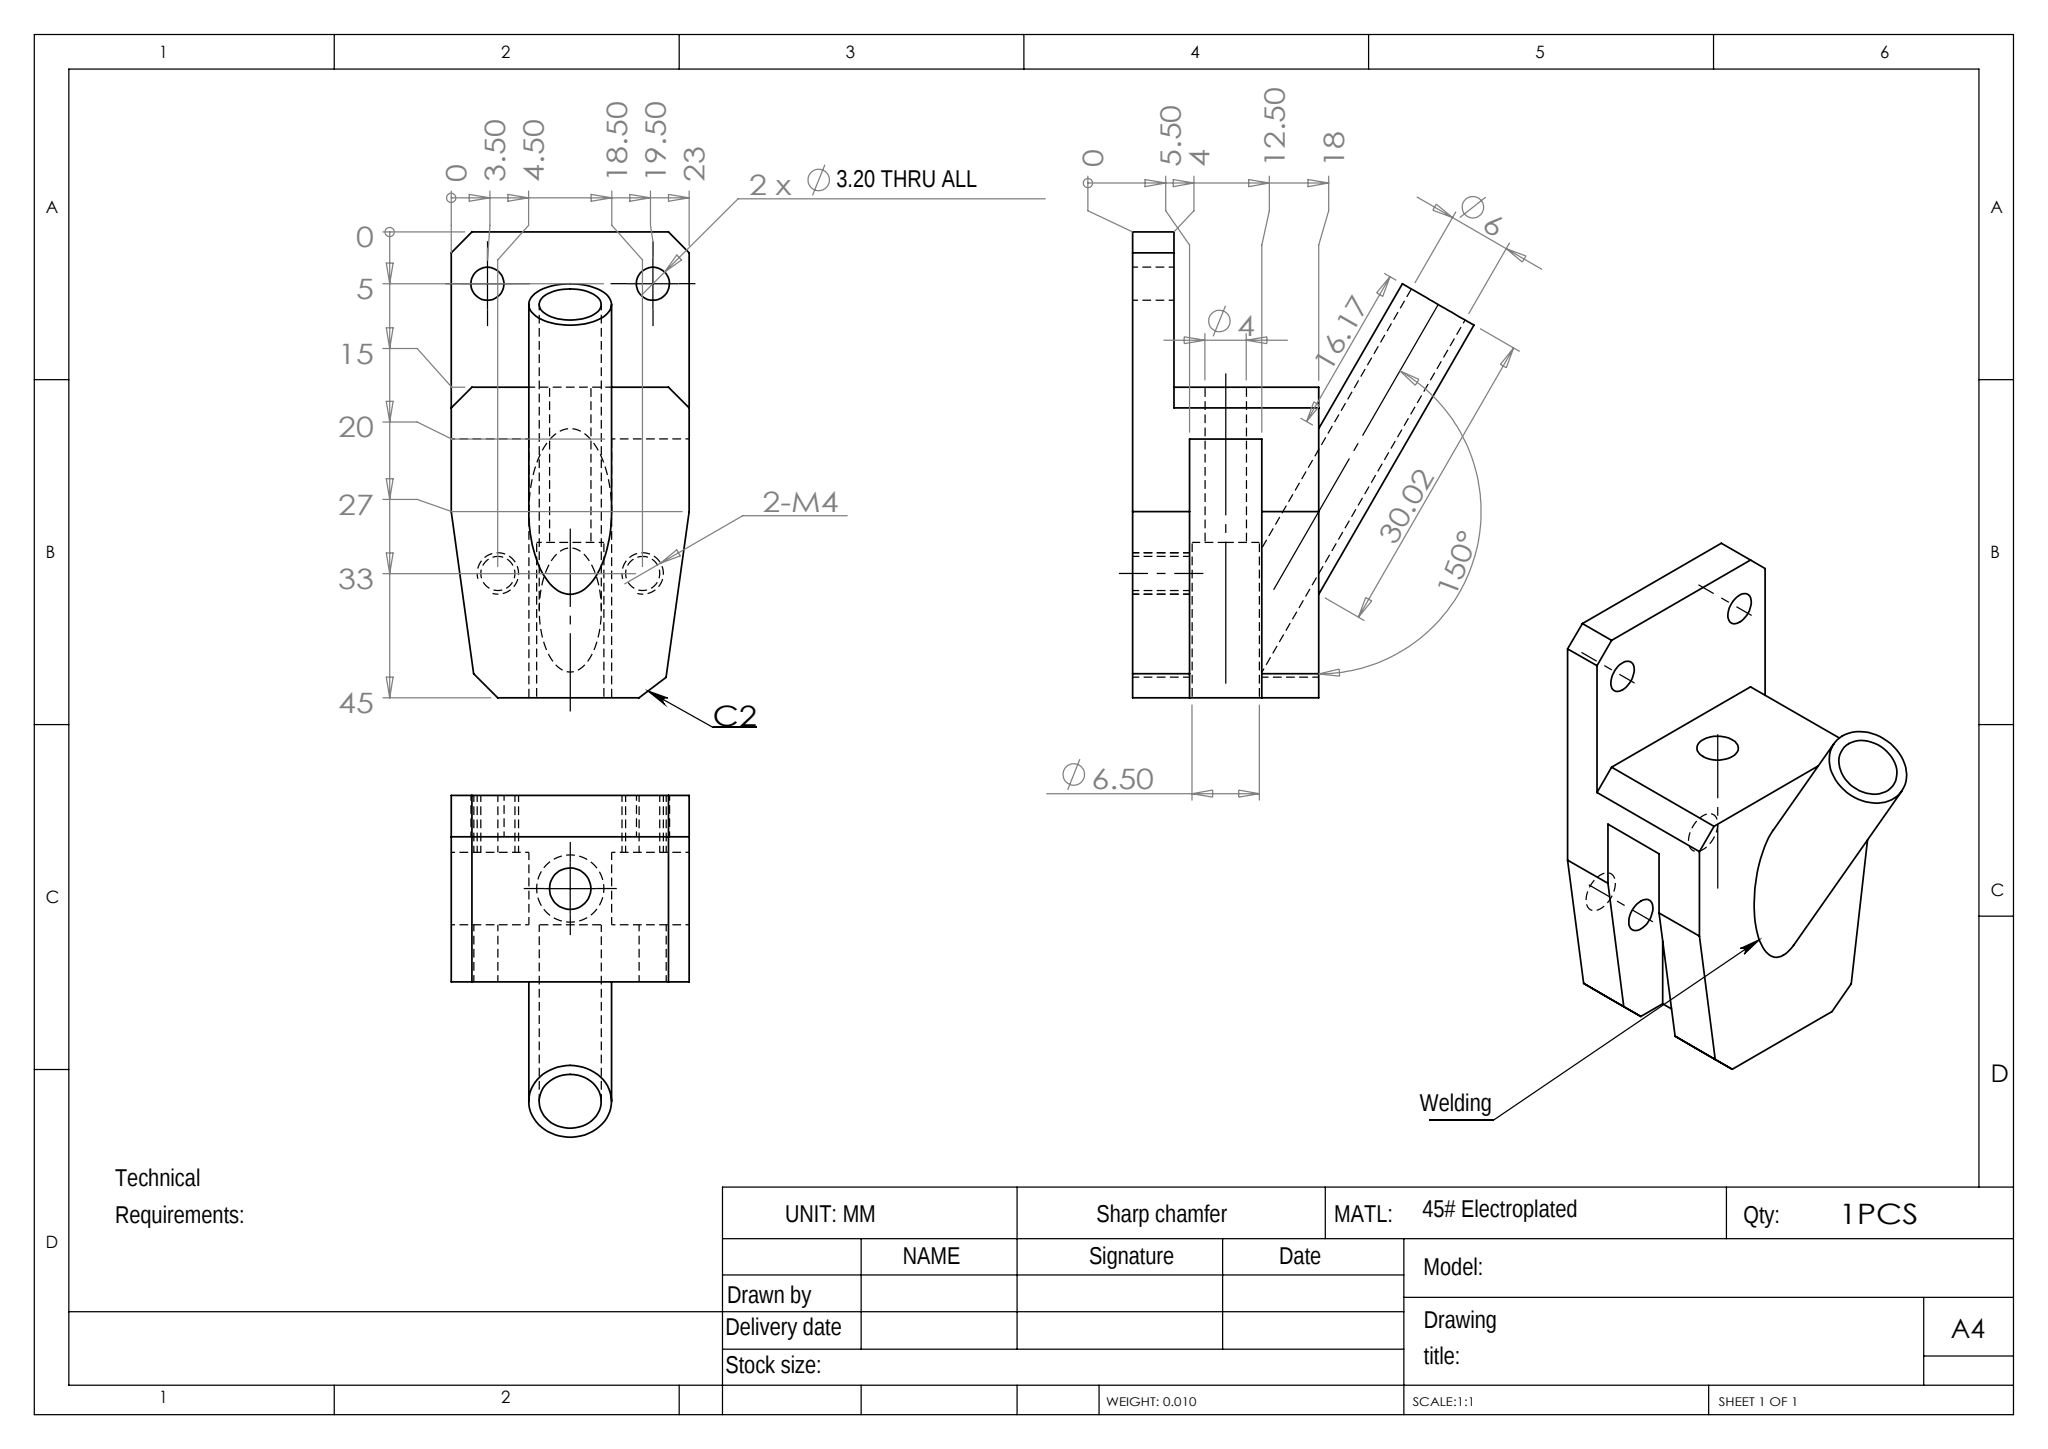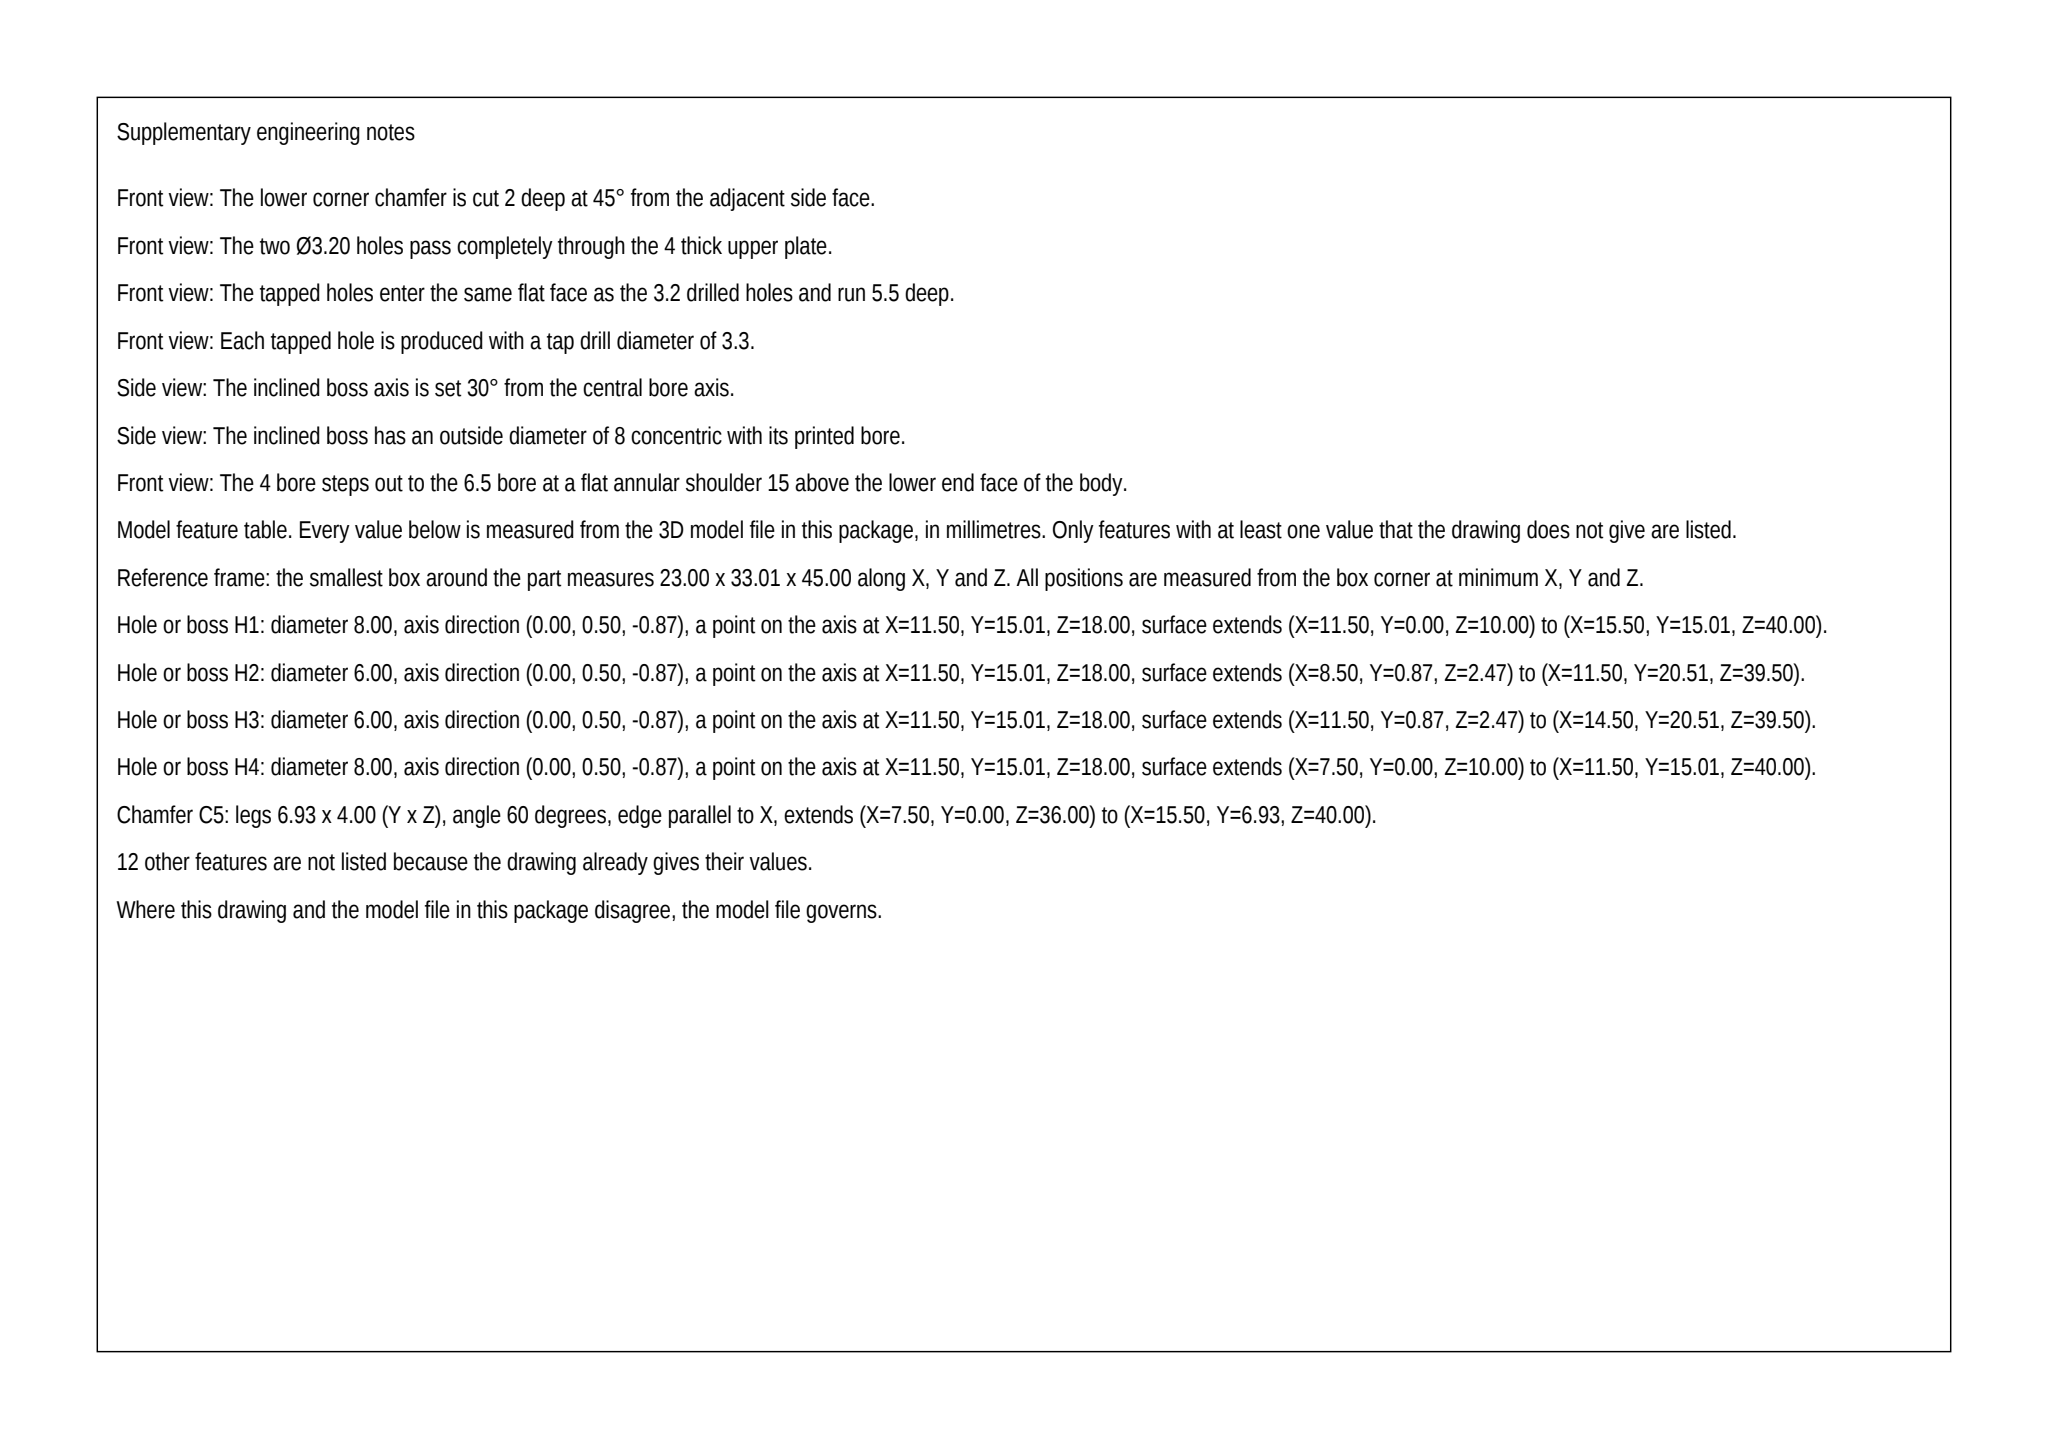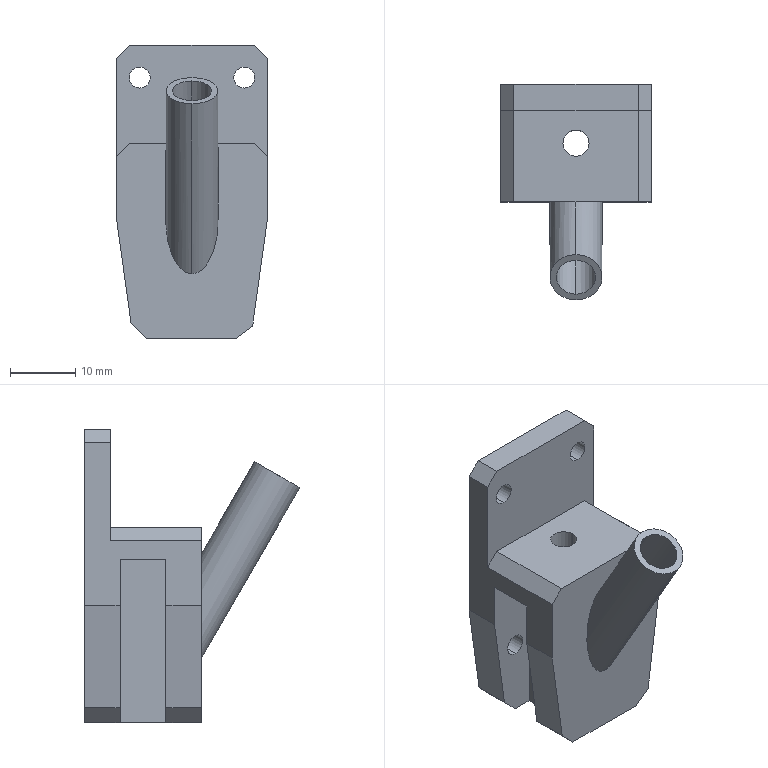Part | SolidWorks | mm | 1 solid | 47 faces | box 23 x 33.01 x 45 mm | volume 9909 mm3 | plane 31 | cylinder 16 | commonest cylinder face diameters 3.2 x4 3.3 x4 4 x2 6.5 x2 8 x2 6 x2